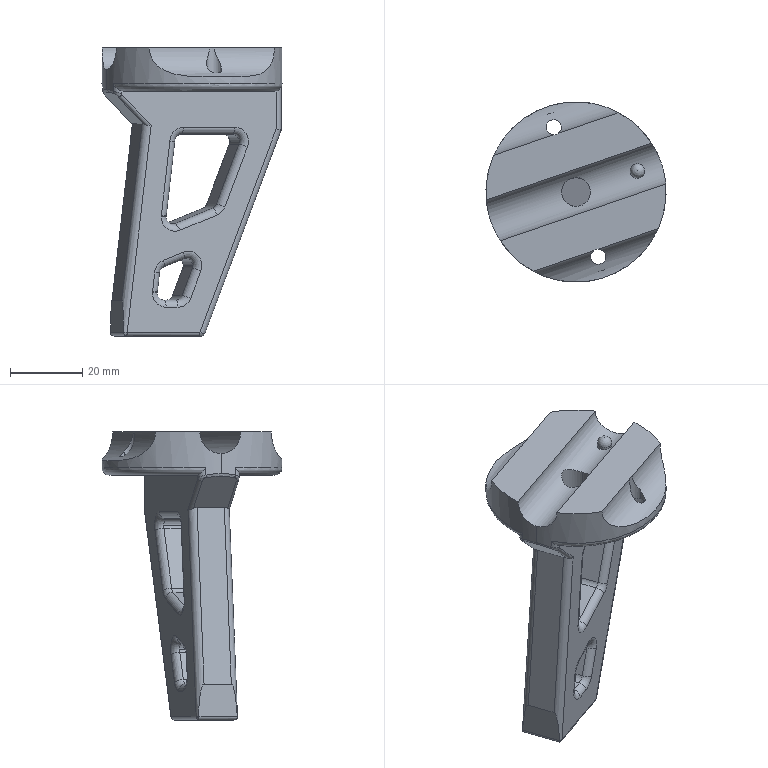Component | SolidWorks | UpperPartOfBracket-3 | 1 solid | 112 faces | volume 39275 mm3 | cylinder 59 | plane 23 | torus 22 | spline 7 | sphere 1 | commonest cylinder face diameters 4 x38 8 x6 2 x6 4.2 x4 50 x2 16 x2 12 x1